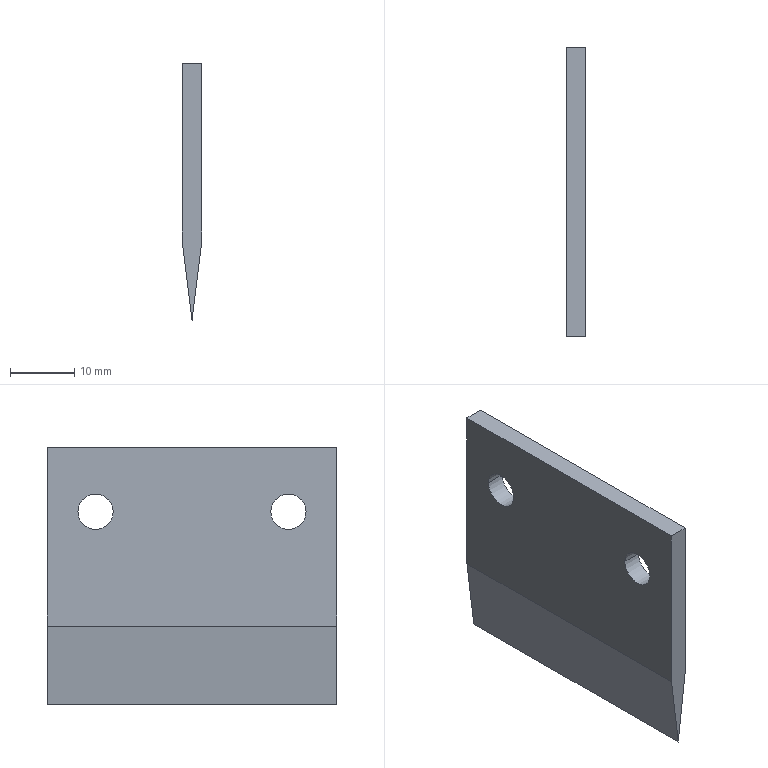Component | SolidWorks | CutterBlade-1 | 1 solid | 11 faces | box 3 x 45 x 40 mm | volume 4433 mm3 | plane 7 | cylinder 4 | commonest cylinder face diameters 5.5 x4 | material Plain Carbon Steel
build123d program:
from build123d import *

# Parameters (mm, degrees)
SKETCH1_W           = 45
SKETCH1_H           = 40
BOSS_EXTRUDE1_DEPTH = 1.5
SKETCH2_R           = 2.75
CUT_EXTRUDE1_DEPTH  = 3
CUT_EXTRUDE2_DEPTH  = 50


with BuildPart() as part:
    # Sketch1 → Boss-Extrude1 (new, symmetric)
    with BuildSketch(Plane.XY):
        with Locations((0, 20)):
            Rectangle(SKETCH1_W, SKETCH1_H)
    extrude(amount=BOSS_EXTRUDE1_DEPTH, both=True)

    # Sketch2 → Cut-Extrude1 (cut)
    with BuildSketch(Plane.XY.offset(1.5)):
        with Locations((-15, 10)):
            Circle(SKETCH2_R)
        with Locations((15, 10)):
            Circle(SKETCH2_R)
    extrude(amount=-CUT_EXTRUDE1_DEPTH, mode=Mode.SUBTRACT)

    # Sketch3 → Cut-Extrude2 (cut, symmetric)
    with BuildSketch(Plane(origin=(0, 0, 0), x_dir=(0, 0, -1), z_dir=(1, 0, 0))):
        Polygon((0, 40), (-1.5, 27.783), (-4.301, 27.783), (-4.301, 45), (3.515, 45), (3.515, 27.783), (1.5, 27.783), align=None)
    extrude(amount=CUT_EXTRUDE2_DEPTH, both=True, mode=Mode.SUBTRACT)


solid = part.part

# Placed as in the assembly
solid = solid.moved(Location((-194.516, 347.264, 141), (-90, 90, 0)))
STEP:
#1=COLOUR_RGB('',0.7922,0.8196,0.9333);
#2=FILL_AREA_STYLE_COLOUR('',#1);
#3=FILL_AREA_STYLE('',(#2));
#4=SURFACE_STYLE_FILL_AREA(#3);
#5=SURFACE_SIDE_STYLE('',(#4));
#6=SURFACE_STYLE_USAGE(.BOTH.,#5);
#7=PRESENTATION_STYLE_ASSIGNMENT((#6));
#8=CARTESIAN_POINT('',(-7.599,14.154,5.157));
#9=VERTEX_POINT('',#8);
#10=CARTESIAN_POINT('',(-7.599,14.371,5.157));
#11=VERTEX_POINT('',#10);
#12=CARTESIAN_POINT('',(-7.599,14.262,5.157));
#13=DIRECTION('',(-1.,0.,-0.));
#14=DIRECTION('',(0.,1.,0.));
#15=AXIS2_PLACEMENT_3D('',#12,#13,#14);
#16=CIRCLE('',#15,0.1083);
#17=EDGE_CURVE('',#9,#11,#16,.T.);
#18=ORIENTED_EDGE('',*,*,#17,.F.);
#19=CARTESIAN_POINT('',(-7.717,14.154,5.157));
#20=VERTEX_POINT('',#19);
#21=CARTESIAN_POINT('',(-7.599,14.154,5.157));
#22=DIRECTION('',(-1.,0.,-0.));
#23=VECTOR('',#22,39.37);
#24=LINE('',#21,#23);
#25=EDGE_CURVE('',#9,#20,#24,.T.);
#26=ORIENTED_EDGE('',*,*,#25,.T.);
#27=CARTESIAN_POINT('',(-7.717,14.371,5.157));
#28=VERTEX_POINT('',#27);
#29=CARTESIAN_POINT('',(-7.717,14.262,5.157));
#30=DIRECTION('',(-1.,0.,-0.));
#31=DIRECTION('',(0.,1.,0.));
#32=AXIS2_PLACEMENT_3D('',#29,#30,#31);
#33=CIRCLE('',#32,0.1083);
#34=EDGE_CURVE('',#20,#28,#33,.T.);
#35=ORIENTED_EDGE('',*,*,#34,.T.);
#36=CARTESIAN_POINT('',(-7.599,14.371,5.157));
#37=DIRECTION('',(-1.,0.,-0.));
#38=VECTOR('',#37,39.37);
#39=LINE('',#36,#38);
#40=EDGE_CURVE('',#11,#28,#39,.T.);
#41=ORIENTED_EDGE('',*,*,#40,.F.);
#42=EDGE_LOOP('',(#18,#26,#35,#41));
#43=FACE_OUTER_BOUND('',#42,.T.);
#44=CARTESIAN_POINT('',(-7.599,14.262,5.157));
#45=DIRECTION('',(-1.,0.,-0.));
#46=DIRECTION('',(0.,1.,0.));
#47=AXIS2_PLACEMENT_3D('',#44,#45,#46);
#48=CYLINDRICAL_SURFACE('',#47,0.1083);
#49=ADVANCED_FACE('',(#43),#48,.F.);
#50=CARTESIAN_POINT('',(-7.599,12.973,5.157));
#51=VERTEX_POINT('',#50);
#52=CARTESIAN_POINT('',(-7.599,13.19,5.157));
#53=VERTEX_POINT('',#52);
#54=CARTESIAN_POINT('',(-7.599,13.081,5.157));
#55=DIRECTION('',(-1.,0.,-0.));
#56=DIRECTION('',(0.,1.,0.));
#57=AXIS2_PLACEMENT_3D('',#54,#55,#56);
#58=CIRCLE('',#57,0.1083);
#59=EDGE_CURVE('',#51,#53,#58,.T.);
#60=ORIENTED_EDGE('',*,*,#59,.F.);
#61=CARTESIAN_POINT('',(-7.717,12.973,5.157));
#62=VERTEX_POINT('',#61);
#63=CARTESIAN_POINT('',(-7.599,12.973,5.157));
#64=DIRECTION('',(-1.,0.,-0.));
#65=VECTOR('',#64,39.37);
#66=LINE('',#63,#65);
#67=EDGE_CURVE('',#51,#62,#66,.T.);
#68=ORIENTED_EDGE('',*,*,#67,.T.);
#69=CARTESIAN_POINT('',(-7.717,13.19,5.157));
#70=VERTEX_POINT('',#69);
#71=CARTESIAN_POINT('',(-7.717,13.081,5.157));
#72=DIRECTION('',(-1.,0.,-0.));
#73=DIRECTION('',(0.,1.,0.));
#74=AXIS2_PLACEMENT_3D('',#71,#72,#73);
#75=CIRCLE('',#74,0.1083);
#76=EDGE_CURVE('',#62,#70,#75,.T.);
#77=ORIENTED_EDGE('',*,*,#76,.T.);
#78=CARTESIAN_POINT('',(-7.599,13.19,5.157));
#79=DIRECTION('',(-1.,0.,-0.));
#80=VECTOR('',#79,39.37);
#81=LINE('',#78,#80);
#82=EDGE_CURVE('',#53,#70,#81,.T.);
#83=ORIENTED_EDGE('',*,*,#82,.F.);
#84=EDGE_LOOP('',(#60,#68,#77,#83));
#85=FACE_OUTER_BOUND('',#84,.T.);
#86=CARTESIAN_POINT('',(-7.599,13.081,5.157));
#87=DIRECTION('',(-1.,0.,-0.));
#88=DIRECTION('',(0.,1.,0.));
#89=AXIS2_PLACEMENT_3D('',#86,#87,#88);
#90=CYLINDRICAL_SURFACE('',#89,0.1083);
#91=ADVANCED_FACE('',(#85),#90,.F.);
#92=CARTESIAN_POINT('',(-7.717,12.786,4.457));
#93=VERTEX_POINT('',#92);
#94=CARTESIAN_POINT('',(-7.658,12.786,3.976));
#95=VERTEX_POINT('',#94);
#96=CARTESIAN_POINT('',(-7.659,12.786,3.984));
#97=DIRECTION('',(0.1219,-0.,-0.9925));
#98=VECTOR('',#97,39.37);
#99=LINE('',#96,#98);
#100=EDGE_CURVE('',#93,#95,#99,.T.);
#101=ORIENTED_EDGE('',*,*,#100,.T.);
#102=CARTESIAN_POINT('',(-7.599,12.786,4.457));
#103=VERTEX_POINT('',#102);
#104=CARTESIAN_POINT('',(-7.659,12.786,3.969));
#105=DIRECTION('',(0.1219,0.,0.9925));
#106=VECTOR('',#105,39.37);
#107=LINE('',#104,#106);
#108=EDGE_CURVE('',#95,#103,#107,.T.);
#109=ORIENTED_EDGE('',*,*,#108,.T.);
#110=CARTESIAN_POINT('',(-7.599,12.786,5.551));
#111=VERTEX_POINT('',#110);
#112=CARTESIAN_POINT('',(-7.599,12.786,3.976));
#113=DIRECTION('',(-0.,0.,1.));
#114=VECTOR('',#113,39.37);
#115=LINE('',#112,#114);
#116=EDGE_CURVE('',#103,#111,#115,.T.);
#117=ORIENTED_EDGE('',*,*,#116,.T.);
#118=CARTESIAN_POINT('',(-7.717,12.786,5.551));
#119=VERTEX_POINT('',#118);
#120=CARTESIAN_POINT('',(-7.717,12.786,5.551));
#121=DIRECTION('',(1.,-0.,0.));
#122=VECTOR('',#121,39.37);
#123=LINE('',#120,#122);
#124=EDGE_CURVE('',#119,#111,#123,.T.);
#125=ORIENTED_EDGE('',*,*,#124,.F.);
#126=CARTESIAN_POINT('',(-7.717,12.786,3.976));
#127=DIRECTION('',(-0.,0.,1.));
#128=VECTOR('',#127,39.37);
#129=LINE('',#126,#128);
#130=EDGE_CURVE('',#93,#119,#129,.T.);
#131=ORIENTED_EDGE('',*,*,#130,.F.);
#132=EDGE_LOOP('',(#101,#109,#117,#125,#131));
#133=FACE_OUTER_BOUND('',#132,.T.);
#134=CARTESIAN_POINT('',(-7.717,12.786,3.976));
#135=DIRECTION('',(0.,1.,-0.));
#136=DIRECTION('',(0.,-0.,-1.));
#137=AXIS2_PLACEMENT_3D('',#134,#135,#136);
#138=PLANE('',#137);
#139=ADVANCED_FACE('',(#133),#138,.F.);
#140=CARTESIAN_POINT('',(-7.599,14.558,5.551));
#141=VERTEX_POINT('',#140);
#142=CARTESIAN_POINT('',(-7.599,12.786,5.551));
#143=DIRECTION('',(0.,1.,-0.));
#144=VECTOR('',#143,39.37);
#145=LINE('',#142,#144);
#146=EDGE_CURVE('',#111,#141,#145,.T.);
#147=ORIENTED_EDGE('',*,*,#146,.T.);
#148=CARTESIAN_POINT('',(-7.717,14.558,5.551));
#149=VERTEX_POINT('',#148);
#150=CARTESIAN_POINT('',(-7.717,14.558,5.551));
#151=DIRECTION('',(1.,-0.,0.));
#152=VECTOR('',#151,39.37);
#153=LINE('',#150,#152);
#154=EDGE_CURVE('',#149,#141,#153,.T.);
#155=ORIENTED_EDGE('',*,*,#154,.F.);
#156=CARTESIAN_POINT('',(-7.717,12.786,5.551));
#157=DIRECTION('',(0.,1.,-0.));
#158=VECTOR('',#157,39.37);
#159=LINE('',#156,#158);
#160=EDGE_CURVE('',#119,#149,#159,.T.);
#161=ORIENTED_EDGE('',*,*,#160,.F.);
#162=ORIENTED_EDGE('',*,*,#124,.T.);
#163=EDGE_LOOP('',(#147,#155,#161,#162));
#164=FACE_OUTER_BOUND('',#163,.T.);
#165=CARTESIAN_POINT('',(-7.717,12.786,5.551));
#166=DIRECTION('',(0.,-0.,-1.));
#167=DIRECTION('',(-1.,0.,-0.));
#168=AXIS2_PLACEMENT_3D('',#165,#166,#167);
#169=PLANE('',#168);
#170=ADVANCED_FACE('',(#164),#169,.F.);
#171=CARTESIAN_POINT('',(-7.599,14.558,4.457));
#172=VERTEX_POINT('',#171);
#173=CARTESIAN_POINT('',(-7.599,14.558,5.551));
#174=DIRECTION('',(0.,-0.,-1.));
#175=VECTOR('',#174,39.37);
#176=LINE('',#173,#175);
#177=EDGE_CURVE('',#141,#172,#176,.T.);
#178=ORIENTED_EDGE('',*,*,#177,.T.);
#179=CARTESIAN_POINT('',(-7.658,14.558,3.976));
#180=VERTEX_POINT('',#179);
#181=CARTESIAN_POINT('',(-7.468,14.558,5.521));
#182=DIRECTION('',(-0.1219,-0.,-0.9925));
#183=VECTOR('',#182,39.37);
#184=LINE('',#181,#183);
#185=EDGE_CURVE('',#172,#180,#184,.T.);
#186=ORIENTED_EDGE('',*,*,#185,.T.);
#187=CARTESIAN_POINT('',(-7.717,14.558,4.457));
#188=VERTEX_POINT('',#187);
#189=CARTESIAN_POINT('',(-7.849,14.558,5.535));
#190=DIRECTION('',(-0.1219,0.,0.9925));
#191=VECTOR('',#190,39.37);
#192=LINE('',#189,#191);
#193=EDGE_CURVE('',#180,#188,#192,.T.);
#194=ORIENTED_EDGE('',*,*,#193,.T.);
#195=CARTESIAN_POINT('',(-7.717,14.558,5.551));
#196=DIRECTION('',(0.,-0.,-1.));
#197=VECTOR('',#196,39.37);
#198=LINE('',#195,#197);
#199=EDGE_CURVE('',#149,#188,#198,.T.);
#200=ORIENTED_EDGE('',*,*,#199,.F.);
#201=ORIENTED_EDGE('',*,*,#154,.T.);
#202=EDGE_LOOP('',(#178,#186,#194,#200,#201));
#203=FACE_OUTER_BOUND('',#202,.T.);
#204=CARTESIAN_POINT('',(-7.717,14.558,5.551));
#205=DIRECTION('',(-0.,-1.,0.));
#206=DIRECTION('',(-0.,0.,1.));
#207=AXIS2_PLACEMENT_3D('',#204,#205,#206);
#208=PLANE('',#207);
#209=ADVANCED_FACE('',(#203),#208,.F.);
#210=CARTESIAN_POINT('',(-7.717,13.672,4.457));
#211=DIRECTION('',(0.,1.,-0.));
#212=VECTOR('',#211,39.37);
#213=LINE('',#210,#212);
#214=EDGE_CURVE('',#93,#188,#213,.T.);
#215=ORIENTED_EDGE('',*,*,#214,.F.);
#216=ORIENTED_EDGE('',*,*,#130,.T.);
#217=ORIENTED_EDGE('',*,*,#160,.T.);
#218=ORIENTED_EDGE('',*,*,#199,.T.);
#219=EDGE_LOOP('',(#215,#216,#217,#218));
#220=FACE_OUTER_BOUND('',#219,.T.);
#221=CARTESIAN_POINT('',(-7.717,14.262,5.157));
#222=DIRECTION('',(-1.,0.,-0.));
#223=DIRECTION('',(0.,1.,0.));
#224=AXIS2_PLACEMENT_3D('',#221,#222,#223);
#225=CIRCLE('',#224,0.1083);
#226=EDGE_CURVE('',#28,#20,#225,.T.);
#227=ORIENTED_EDGE('',*,*,#226,.F.);
#228=ORIENTED_EDGE('',*,*,#34,.F.);
#229=EDGE_LOOP('',(#227,#228));
#230=FACE_BOUND('',#229,.T.);
#231=CARTESIAN_POINT('',(-7.717,13.081,5.157));
#232=DIRECTION('',(-1.,0.,-0.));
#233=DIRECTION('',(0.,1.,0.));
#234=AXIS2_PLACEMENT_3D('',#231,#232,#233);
#235=CIRCLE('',#234,0.1083);
#236=EDGE_CURVE('',#70,#62,#235,.T.);
#237=ORIENTED_EDGE('',*,*,#236,.F.);
#238=ORIENTED_EDGE('',*,*,#76,.F.);
#239=EDGE_LOOP('',(#237,#238));
#240=FACE_BOUND('',#239,.T.);
#241=CARTESIAN_POINT('',(-7.717,13.672,5.551));
#242=DIRECTION('',(-1.,0.,-0.));
#243=DIRECTION('',(0.,1.,-0.));
#244=AXIS2_PLACEMENT_3D('',#241,#242,#243);
#245=PLANE('',#244);
#246=ADVANCED_FACE('',(#220,#230,#240),#245,.T.);
#247=CARTESIAN_POINT('',(-7.599,14.262,5.157));
#248=DIRECTION('',(-1.,0.,-0.));
#249=DIRECTION('',(0.,1.,0.));
#250=AXIS2_PLACEMENT_3D('',#247,#248,#249);
#251=CIRCLE('',#250,0.1083);
#252=EDGE_CURVE('',#11,#9,#251,.T.);
#253=ORIENTED_EDGE('',*,*,#252,.T.);
#254=ORIENTED_EDGE('',*,*,#17,.T.);
#255=EDGE_LOOP('',(#253,#254));
#256=FACE_BOUND('',#255,.T.);
#257=CARTESIAN_POINT('',(-7.599,13.081,5.157));
#258=DIRECTION('',(-1.,0.,-0.));
#259=DIRECTION('',(0.,1.,0.));
#260=AXIS2_PLACEMENT_3D('',#257,#258,#259);
#261=CIRCLE('',#260,0.1083);
#262=EDGE_CURVE('',#53,#51,#261,.T.);
#263=ORIENTED_EDGE('',*,*,#262,.T.);
#264=ORIENTED_EDGE('',*,*,#59,.T.);
#265=EDGE_LOOP('',(#263,#264));
#266=FACE_BOUND('',#265,.T.);
#267=ORIENTED_EDGE('',*,*,#116,.F.);
#268=CARTESIAN_POINT('',(-7.599,13.672,4.457));
#269=DIRECTION('',(0.,1.,-0.));
#270=VECTOR('',#269,39.37);
#271=LINE('',#268,#270);
#272=EDGE_CURVE('',#103,#172,#271,.T.);
#273=ORIENTED_EDGE('',*,*,#272,.T.);
#274=ORIENTED_EDGE('',*,*,#177,.F.);
#275=ORIENTED_EDGE('',*,*,#146,.F.);
#276=EDGE_LOOP('',(#267,#273,#274,#275));
#277=FACE_OUTER_BOUND('',#276,.T.);
#278=CARTESIAN_POINT('',(-7.599,13.672,5.551));
#279=DIRECTION('',(-1.,0.,-0.));
#280=DIRECTION('',(0.,1.,-0.));
#281=AXIS2_PLACEMENT_3D('',#278,#279,#280);
#282=PLANE('',#281);
#283=ADVANCED_FACE('',(#256,#266,#277),#282,.F.);
#284=ORIENTED_EDGE('',*,*,#67,.F.);
#285=ORIENTED_EDGE('',*,*,#262,.F.);
#286=ORIENTED_EDGE('',*,*,#82,.T.);
#287=ORIENTED_EDGE('',*,*,#236,.T.);
#288=EDGE_LOOP('',(#284,#285,#286,#287));
#289=FACE_OUTER_BOUND('',#288,.T.);
#290=CARTESIAN_POINT('',(-7.599,13.081,5.157));
#291=DIRECTION('',(-1.,0.,-0.));
#292=DIRECTION('',(0.,1.,0.));
#293=AXIS2_PLACEMENT_3D('',#290,#291,#292);
#294=CYLINDRICAL_SURFACE('',#293,0.1083);
#295=ADVANCED_FACE('',(#289),#294,.F.);
#296=ORIENTED_EDGE('',*,*,#25,.F.);
#297=ORIENTED_EDGE('',*,*,#252,.F.);
#298=ORIENTED_EDGE('',*,*,#40,.T.);
#299=ORIENTED_EDGE('',*,*,#226,.T.);
#300=EDGE_LOOP('',(#296,#297,#298,#299));
#301=FACE_OUTER_BOUND('',#300,.T.);
#302=CARTESIAN_POINT('',(-7.599,14.262,5.157));
#303=DIRECTION('',(-1.,0.,-0.));
#304=DIRECTION('',(0.,1.,0.));
#305=AXIS2_PLACEMENT_3D('',#302,#303,#304);
#306=CYLINDRICAL_SURFACE('',#305,0.1083);
#307=ADVANCED_FACE('',(#301),#306,.F.);
#308=ORIENTED_EDGE('',*,*,#214,.T.);
#309=ORIENTED_EDGE('',*,*,#193,.F.);
#310=CARTESIAN_POINT('',(-7.658,11.703,3.976));
#311=DIRECTION('',(0.,1.,-0.));
#312=VECTOR('',#311,39.37);
#313=LINE('',#310,#312);
#314=EDGE_CURVE('',#95,#180,#313,.T.);
#315=ORIENTED_EDGE('',*,*,#314,.F.);
#316=ORIENTED_EDGE('',*,*,#100,.F.);
#317=EDGE_LOOP('',(#308,#309,#315,#316));
#318=FACE_OUTER_BOUND('',#317,.T.);
#319=CARTESIAN_POINT('',(-7.658,11.703,3.976));
#320=DIRECTION('',(0.9925,0.,0.1219));
#321=DIRECTION('',(0.1219,-0.,-0.9925));
#322=AXIS2_PLACEMENT_3D('',#319,#320,#321);
#323=PLANE('',#322);
#324=ADVANCED_FACE('',(#318),#323,.F.);
#325=ORIENTED_EDGE('',*,*,#314,.T.);
#326=ORIENTED_EDGE('',*,*,#185,.F.);
#327=ORIENTED_EDGE('',*,*,#272,.F.);
#328=ORIENTED_EDGE('',*,*,#108,.F.);
#329=EDGE_LOOP('',(#325,#326,#327,#328));
#330=FACE_OUTER_BOUND('',#329,.T.);
#331=CARTESIAN_POINT('',(-7.658,11.703,3.976));
#332=DIRECTION('',(-0.9925,0.,0.1219));
#333=DIRECTION('',(0.1219,0.,0.9925));
#334=AXIS2_PLACEMENT_3D('',#331,#332,#333);
#335=PLANE('',#334);
#336=ADVANCED_FACE('',(#330),#335,.F.);
#337=CLOSED_SHELL('',(#49,#91,#139,#170,#209,#246,#283,#295,#307,#324,#336));
#338=MANIFOLD_SOLID_BREP('',#337);
#339=STYLED_ITEM('',(#7),#338);
#340=(LENGTH_UNIT()NAMED_UNIT(*)SI_UNIT($,.METRE.));
#341=LENGTH_MEASURE_WITH_UNIT(LENGTH_MEASURE(0.0254),#340);
#342=DIMENSIONAL_EXPONENTS(1.,0.,0.,0.,0.,0.,0.);
#343=(CONVERSION_BASED_UNIT('',#341)LENGTH_UNIT()NAMED_UNIT(#342));
#344=UNCERTAINTY_MEASURE_WITH_UNIT(LENGTH_MEASURE(0.00001),#343,'','');
#345=(NAMED_UNIT(*)PLANE_ANGLE_UNIT()SI_UNIT($,.RADIAN.));
#346=(NAMED_UNIT(*)SI_UNIT($,.STERADIAN.)SOLID_ANGLE_UNIT());
#347=(GEOMETRIC_REPRESENTATION_CONTEXT(3)GLOBAL_UNCERTAINTY_ASSIGNED_CONTEXT((#344))GLOBAL_UNIT_ASSIGNED_CONTEXT((#343,#345,#346))REPRESENTATION_CONTEXT('',''));
#348=MECHANICAL_DESIGN_GEOMETRIC_PRESENTATION_REPRESENTATION('',(#339),#347);
#349=PRESENTATION_LAYER_ASSIGNMENT('','',(#339));
#350=CARTESIAN_POINT('',(0.,0.,0.));
#351=DIRECTION('',(0.,0.,1.));
#352=DIRECTION('',(1.,0.,0.));
#353=AXIS2_PLACEMENT_3D('',#350,#351,#352);
#354=(LENGTH_UNIT()NAMED_UNIT(*)SI_UNIT($,.METRE.));
#355=LENGTH_MEASURE_WITH_UNIT(LENGTH_MEASURE(0.0254),#354);
#356=DIMENSIONAL_EXPONENTS(1.,0.,0.,0.,0.,0.,0.);
#357=(CONVERSION_BASED_UNIT('',#355)LENGTH_UNIT()NAMED_UNIT(#356));
#358=UNCERTAINTY_MEASURE_WITH_UNIT(LENGTH_MEASURE(0.00001),#357,'','');
#359=(NAMED_UNIT(*)PLANE_ANGLE_UNIT()SI_UNIT($,.RADIAN.));
#360=(NAMED_UNIT(*)SI_UNIT($,.STERADIAN.)SOLID_ANGLE_UNIT());
#361=(GEOMETRIC_REPRESENTATION_CONTEXT(3)GLOBAL_UNCERTAINTY_ASSIGNED_CONTEXT((#358))GLOBAL_UNIT_ASSIGNED_CONTEXT((#357,#359,#360))REPRESENTATION_CONTEXT('',''));
#362=ADVANCED_BREP_SHAPE_REPRESENTATION('',(#338,#353),#361);